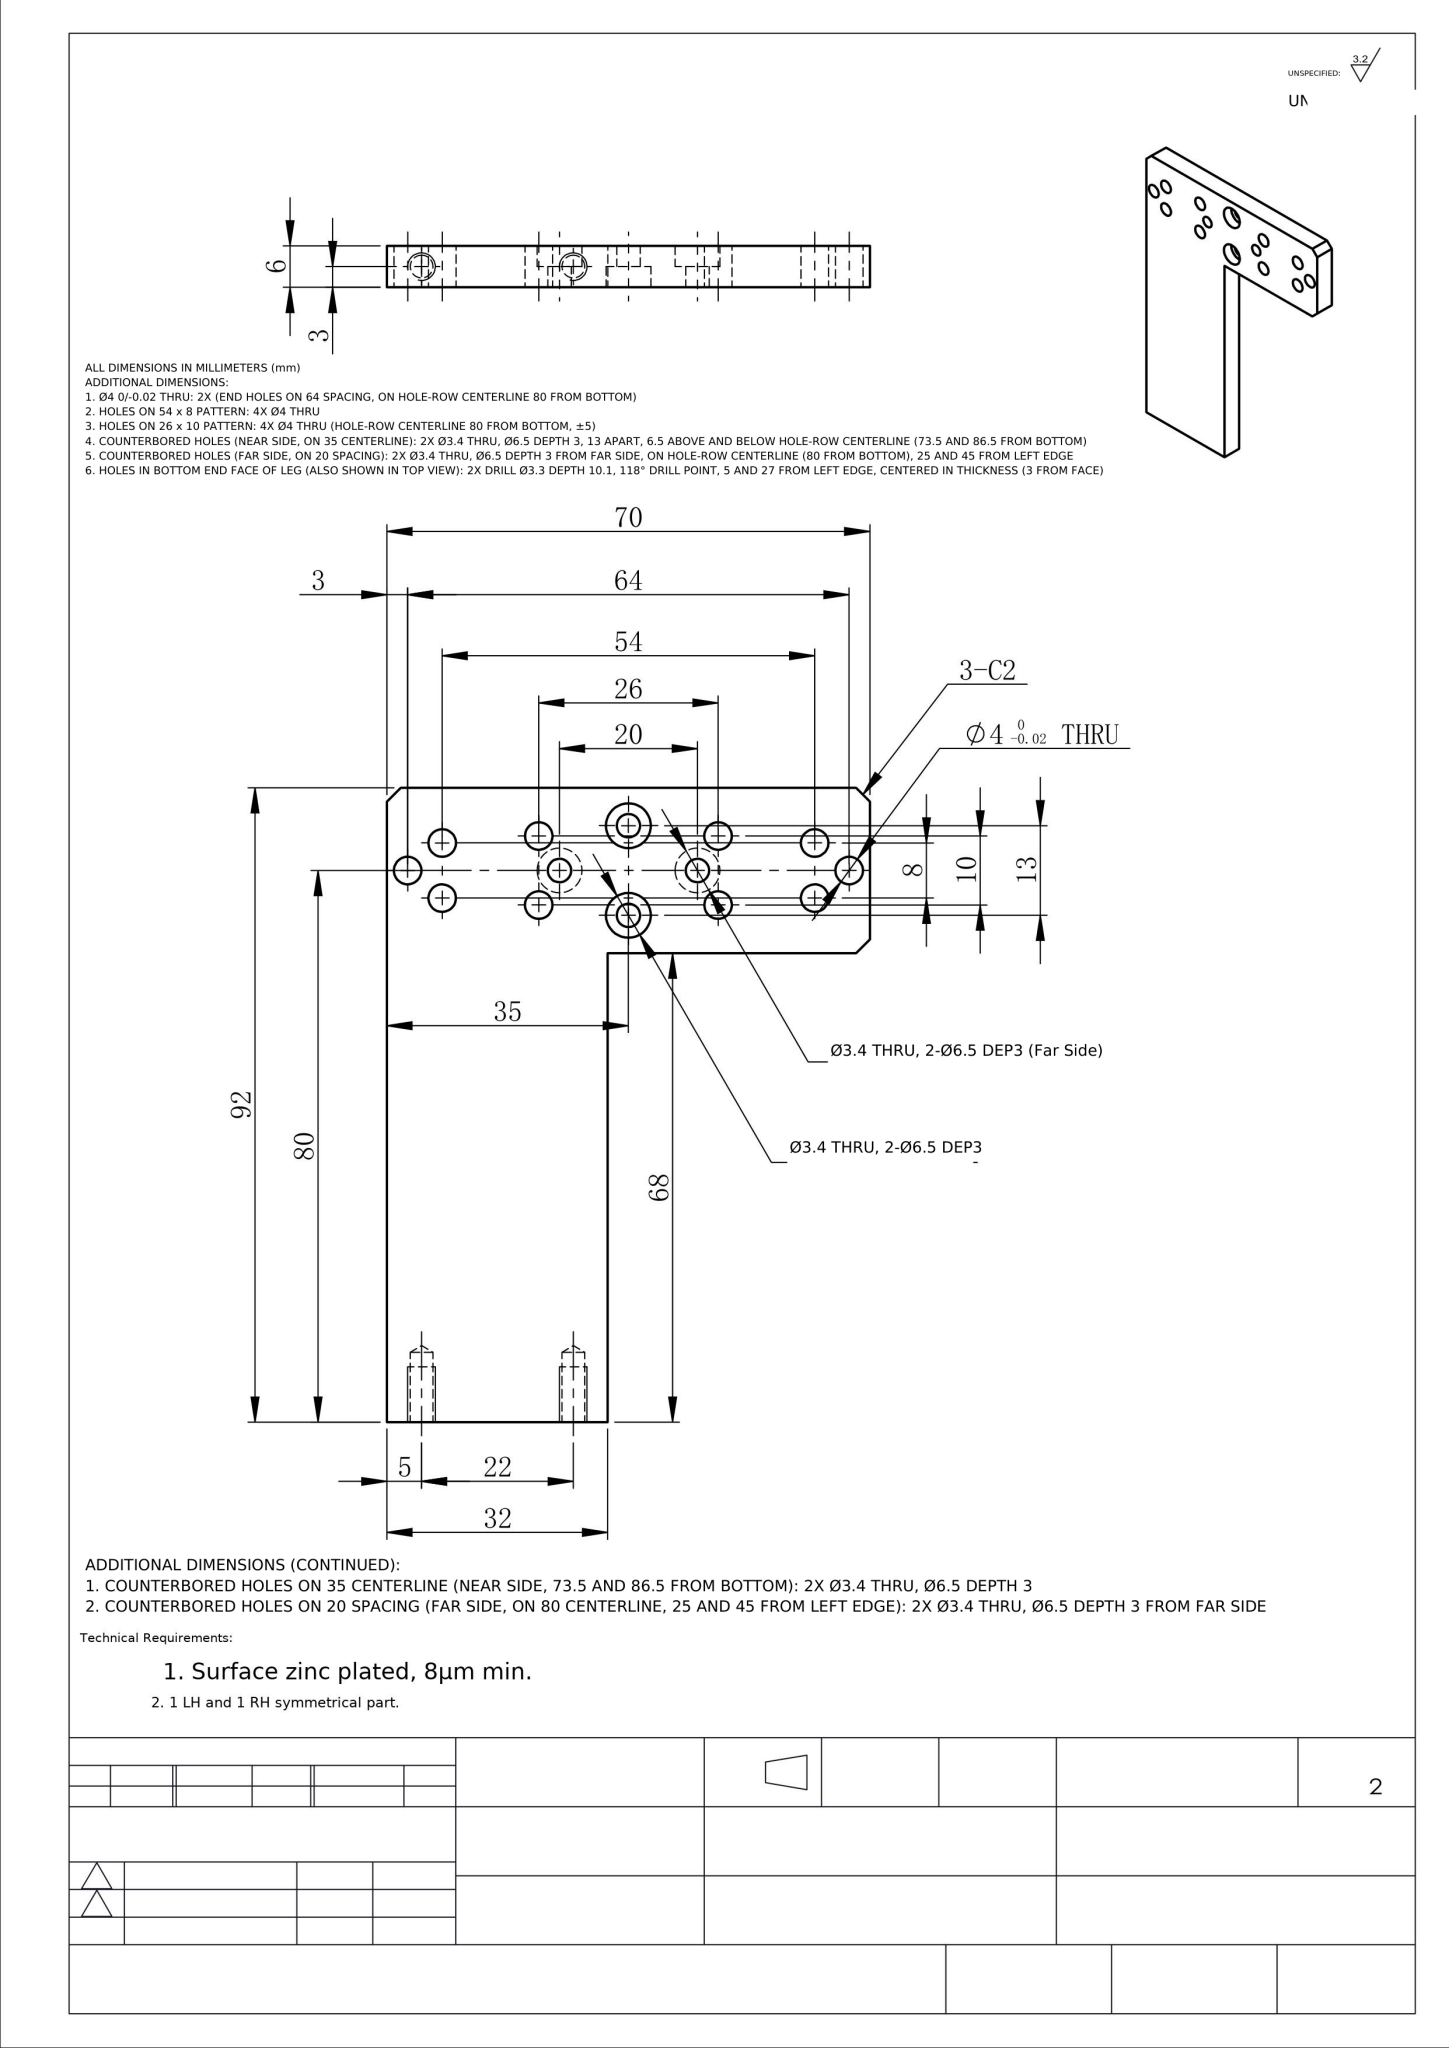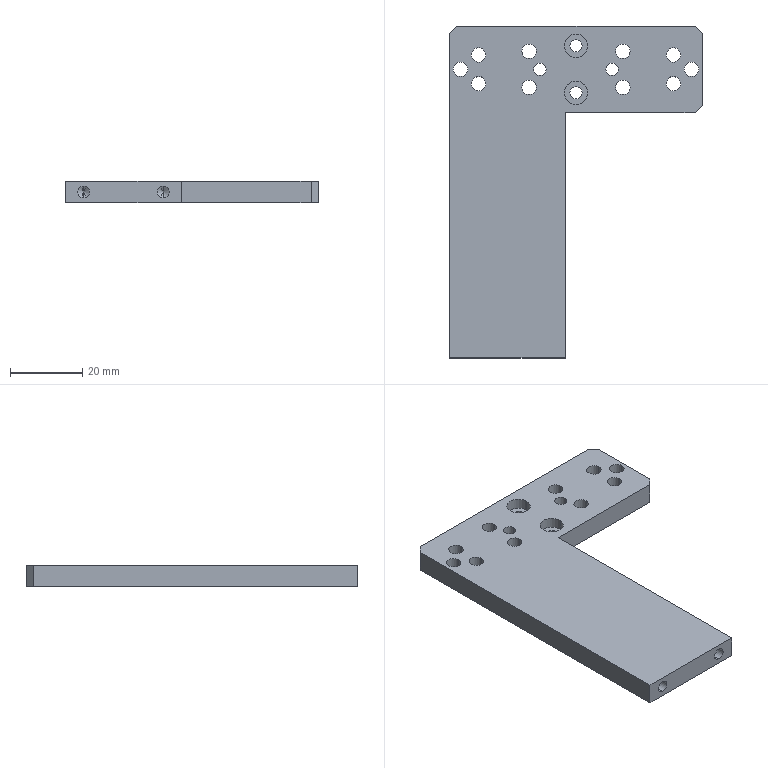Part | NX | mm | 1 solid | 59 faces | box 70 x 92 x 6 mm | volume 21660 mm3 | cylinder 40 | plane 15 | cone 4 | commonest cylinder face diameters 4 x20 3.4 x8 6.5 x8 3.3 x4